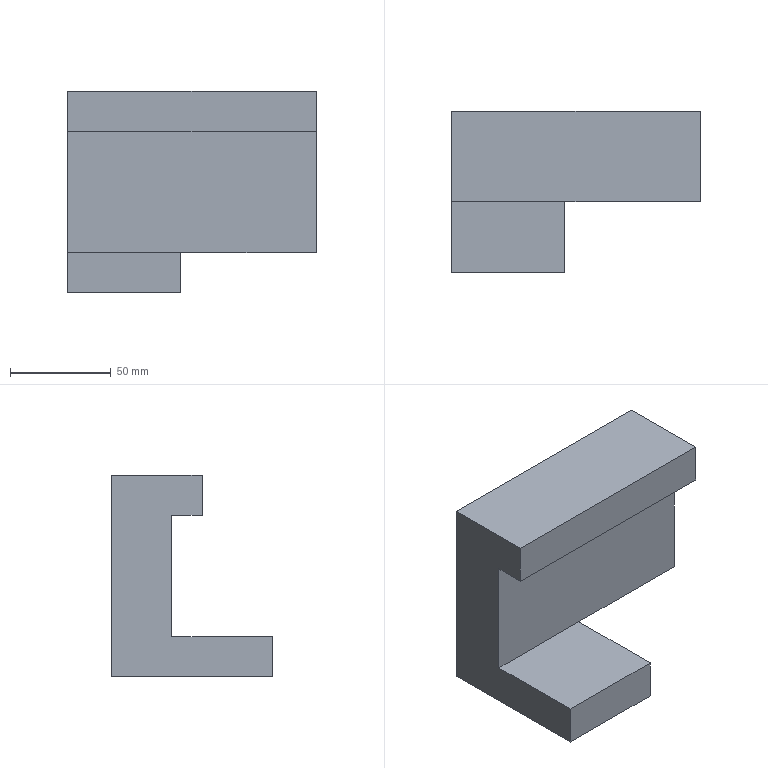Component | SolidWorks | ParallelGripperFingerA-1 | 1 solid | 12 faces | box 123 x 80 x 100 mm | volume 421700 mm3 | plane 12 | material Aviation Aluminum-7075
build123d program:
from build123d import *

# Parameters (mm, degrees)
SKETCH1_W           = 80
SKETCH1_H           = 56
BOSS_EXTRUDE1_DEPTH = 20
SKETCH2_W           = 30
SKETCH2_H           = 56
BOSS_EXTRUDE2_DEPTH = 80
SKETCH3_W           = 30
SKETCH3_H           = 80
BOSS_EXTRUDE3_DEPTH = 67
SKETCH4_W           = 20
SKETCH4_H           = 123
BOSS_EXTRUDE4_DEPTH = 15


with BuildPart() as part:
    # Sketch1 → Boss-Extrude1 (new body)
    with BuildSketch(Plane.XY):
        Rectangle(SKETCH1_W, SKETCH1_H)
    extrude(amount=BOSS_EXTRUDE1_DEPTH)

    # Sketch2 → Boss-Extrude2 (add)
    with BuildSketch(Plane.XY.offset(20)):
        with Locations((25, 0)):
            Rectangle(SKETCH2_W, SKETCH2_H)
    extrude(amount=BOSS_EXTRUDE2_DEPTH)

    # Sketch3 → Boss-Extrude3 (add)
    with BuildSketch(Plane(origin=(0, -28, 0), x_dir=(1, 0, 0), z_dir=(0, 1, 0))):
        with Locations((25, -60)):
            Rectangle(SKETCH3_W, SKETCH3_H)
    extrude(amount=-BOSS_EXTRUDE3_DEPTH)

    # Sketch4 → Boss-Extrude4 (add)
    with BuildSketch(Plane.ZY.offset(-10)):
        with Locations((90, -33.5)):
            Rectangle(SKETCH4_W, SKETCH4_H)
    extrude(amount=BOSS_EXTRUDE4_DEPTH)


solid = part.part

# Placed as in the assembly
solid = solid.moved(Location((-80.87, -240.626, 497.215), (0, 0, 90)))
STEP:
#1=CARTESIAN_POINT('',(-4.286,-9.08,22.725));
#2=VERTEX_POINT('',#1);
#3=CARTESIAN_POINT('',(0.5563,-9.08,22.725));
#4=VERTEX_POINT('',#3);
#5=CARTESIAN_POINT('',(0.5563,-9.08,22.725));
#6=DIRECTION('',(1.,0.,0.));
#7=VECTOR('',#6,39.37);
#8=LINE('',#5,#7);
#9=EDGE_CURVE('',#2,#4,#8,.T.);
#10=ORIENTED_EDGE('',*,*,#9,.F.);
#11=CARTESIAN_POINT('',(-4.286,-9.08,20.363));
#12=VERTEX_POINT('',#11);
#13=CARTESIAN_POINT('',(-4.286,-9.08,23.512));
#14=DIRECTION('',(0.,0.,-1.));
#15=VECTOR('',#14,39.37);
#16=LINE('',#13,#15);
#17=EDGE_CURVE('',#2,#12,#16,.T.);
#18=ORIENTED_EDGE('',*,*,#17,.T.);
#19=CARTESIAN_POINT('',(-2.081,-9.08,20.363));
#20=VERTEX_POINT('',#19);
#21=CARTESIAN_POINT('',(-4.286,-9.08,20.363));
#22=DIRECTION('',(1.,0.,0.));
#23=VECTOR('',#22,39.37);
#24=LINE('',#21,#23);
#25=EDGE_CURVE('',#12,#20,#24,.T.);
#26=ORIENTED_EDGE('',*,*,#25,.T.);
#27=CARTESIAN_POINT('',(0.5563,-9.08,20.363));
#28=VERTEX_POINT('',#27);
#29=CARTESIAN_POINT('',(0.5563,-9.08,20.363));
#30=DIRECTION('',(-1.,-0.,0.));
#31=VECTOR('',#30,39.37);
#32=LINE('',#29,#31);
#33=EDGE_CURVE('',#28,#20,#32,.T.);
#34=ORIENTED_EDGE('',*,*,#33,.F.);
#35=CARTESIAN_POINT('',(0.5563,-9.08,20.363));
#36=DIRECTION('',(0.,0.,1.));
#37=VECTOR('',#36,39.37);
#38=LINE('',#35,#37);
#39=EDGE_CURVE('',#28,#4,#38,.T.);
#40=ORIENTED_EDGE('',*,*,#39,.T.);
#41=EDGE_LOOP('',(#10,#18,#26,#34,#40));
#42=FACE_OUTER_BOUND('',#41,.T.);
#43=CARTESIAN_POINT('',(-4.286,-9.08,23.512));
#44=DIRECTION('',(-0.,1.,0.));
#45=DIRECTION('',(-1.,-0.,0.));
#46=AXIS2_PLACEMENT_3D('',#43,#44,#45);
#47=PLANE('',#46);
#48=ADVANCED_FACE('',(#42),#47,.F.);
#49=CARTESIAN_POINT('',(-4.286,-11.048,19.575));
#50=VERTEX_POINT('',#49);
#51=CARTESIAN_POINT('',(-2.081,-11.048,19.575));
#52=VERTEX_POINT('',#51);
#53=CARTESIAN_POINT('',(-2.081,-11.048,19.575));
#54=DIRECTION('',(1.,-0.,0.));
#55=VECTOR('',#54,39.37);
#56=LINE('',#53,#55);
#57=EDGE_CURVE('',#50,#52,#56,.T.);
#58=ORIENTED_EDGE('',*,*,#57,.T.);
#59=CARTESIAN_POINT('',(-2.081,-11.048,20.363));
#60=VERTEX_POINT('',#59);
#61=CARTESIAN_POINT('',(-2.081,-11.048,20.363));
#62=DIRECTION('',(0.,0.,-1.));
#63=VECTOR('',#62,39.37);
#64=LINE('',#61,#63);
#65=EDGE_CURVE('',#60,#52,#64,.T.);
#66=ORIENTED_EDGE('',*,*,#65,.F.);
#67=CARTESIAN_POINT('',(-4.286,-11.048,20.363));
#68=VERTEX_POINT('',#67);
#69=CARTESIAN_POINT('',(-2.081,-11.048,20.363));
#70=DIRECTION('',(1.,-0.,0.));
#71=VECTOR('',#70,39.37);
#72=LINE('',#69,#71);
#73=EDGE_CURVE('',#68,#60,#72,.T.);
#74=ORIENTED_EDGE('',*,*,#73,.F.);
#75=CARTESIAN_POINT('',(-4.286,-11.048,20.363));
#76=DIRECTION('',(0.,0.,-1.));
#77=VECTOR('',#76,39.37);
#78=LINE('',#75,#77);
#79=EDGE_CURVE('',#68,#50,#78,.T.);
#80=ORIENTED_EDGE('',*,*,#79,.T.);
#81=EDGE_LOOP('',(#58,#66,#74,#80));
#82=FACE_OUTER_BOUND('',#81,.T.);
#83=CARTESIAN_POINT('',(-2.081,-11.048,20.363));
#84=DIRECTION('',(0.,1.,0.));
#85=DIRECTION('',(0.,0.,-1.));
#86=AXIS2_PLACEMENT_3D('',#83,#84,#85);
#87=PLANE('',#86);
#88=ADVANCED_FACE('',(#82),#87,.F.);
#89=CARTESIAN_POINT('',(-2.081,-7.899,20.363));
#90=VERTEX_POINT('',#89);
#91=CARTESIAN_POINT('',(-2.081,-7.899,19.575));
#92=VERTEX_POINT('',#91);
#93=CARTESIAN_POINT('',(-2.081,-7.899,20.363));
#94=DIRECTION('',(0.,0.,-1.));
#95=VECTOR('',#94,39.37);
#96=LINE('',#93,#95);
#97=EDGE_CURVE('',#90,#92,#96,.T.);
#98=ORIENTED_EDGE('',*,*,#97,.F.);
#99=CARTESIAN_POINT('',(-2.081,-9.08,20.363));
#100=DIRECTION('',(0.,-1.,0.));
#101=VECTOR('',#100,39.37);
#102=LINE('',#99,#101);
#103=EDGE_CURVE('',#90,#20,#102,.T.);
#104=ORIENTED_EDGE('',*,*,#103,.T.);
#105=CARTESIAN_POINT('',(-2.081,-7.899,20.363));
#106=DIRECTION('',(-0.,1.,0.));
#107=VECTOR('',#106,39.37);
#108=LINE('',#105,#107);
#109=EDGE_CURVE('',#60,#20,#108,.T.);
#110=ORIENTED_EDGE('',*,*,#109,.F.);
#111=ORIENTED_EDGE('',*,*,#65,.T.);
#112=CARTESIAN_POINT('',(-2.081,-7.899,19.575));
#113=DIRECTION('',(-0.,1.,0.));
#114=VECTOR('',#113,39.37);
#115=LINE('',#112,#114);
#116=EDGE_CURVE('',#52,#92,#115,.T.);
#117=ORIENTED_EDGE('',*,*,#116,.T.);
#118=EDGE_LOOP('',(#98,#104,#110,#111,#117));
#119=FACE_OUTER_BOUND('',#118,.T.);
#120=CARTESIAN_POINT('',(-2.081,-7.899,20.363));
#121=DIRECTION('',(-1.,-0.,0.));
#122=DIRECTION('',(0.,-1.,0.));
#123=AXIS2_PLACEMENT_3D('',#120,#121,#122);
#124=PLANE('',#123);
#125=ADVANCED_FACE('',(#119),#124,.F.);
#126=CARTESIAN_POINT('',(-4.286,-7.899,19.575));
#127=VERTEX_POINT('',#126);
#128=CARTESIAN_POINT('',(-2.081,-7.899,19.575));
#129=DIRECTION('',(-1.,0.,0.));
#130=VECTOR('',#129,39.37);
#131=LINE('',#128,#130);
#132=EDGE_CURVE('',#92,#127,#131,.T.);
#133=ORIENTED_EDGE('',*,*,#132,.T.);
#134=CARTESIAN_POINT('',(-4.286,-7.899,23.512));
#135=VERTEX_POINT('',#134);
#136=CARTESIAN_POINT('',(-4.286,-7.899,20.363));
#137=DIRECTION('',(0.,0.,-1.));
#138=VECTOR('',#137,39.37);
#139=LINE('',#136,#138);
#140=EDGE_CURVE('',#135,#127,#139,.T.);
#141=ORIENTED_EDGE('',*,*,#140,.F.);
#142=CARTESIAN_POINT('',(0.5563,-7.899,23.512));
#143=VERTEX_POINT('',#142);
#144=CARTESIAN_POINT('',(-4.286,-7.899,23.512));
#145=DIRECTION('',(-1.,0.,0.));
#146=VECTOR('',#145,39.37);
#147=LINE('',#144,#146);
#148=EDGE_CURVE('',#143,#135,#147,.T.);
#149=ORIENTED_EDGE('',*,*,#148,.F.);
#150=CARTESIAN_POINT('',(0.5563,-7.899,20.363));
#151=VERTEX_POINT('',#150);
#152=CARTESIAN_POINT('',(0.5563,-7.899,20.363));
#153=DIRECTION('',(0.,0.,-1.));
#154=VECTOR('',#153,39.37);
#155=LINE('',#152,#154);
#156=EDGE_CURVE('',#143,#151,#155,.T.);
#157=ORIENTED_EDGE('',*,*,#156,.T.);
#158=CARTESIAN_POINT('',(0.5563,-7.899,20.363));
#159=DIRECTION('',(-1.,-0.,0.));
#160=VECTOR('',#159,39.37);
#161=LINE('',#158,#160);
#162=EDGE_CURVE('',#151,#90,#161,.T.);
#163=ORIENTED_EDGE('',*,*,#162,.T.);
#164=ORIENTED_EDGE('',*,*,#97,.T.);
#165=EDGE_LOOP('',(#133,#141,#149,#157,#163,#164));
#166=FACE_OUTER_BOUND('',#165,.T.);
#167=CARTESIAN_POINT('',(-2.081,-7.899,20.363));
#168=DIRECTION('',(-0.,-1.,0.));
#169=DIRECTION('',(0.,0.,1.));
#170=AXIS2_PLACEMENT_3D('',#167,#168,#169);
#171=PLANE('',#170);
#172=ADVANCED_FACE('',(#166),#171,.F.);
#173=CARTESIAN_POINT('',(-4.286,-7.899,19.575));
#174=DIRECTION('',(0.,-1.,0.));
#175=VECTOR('',#174,39.37);
#176=LINE('',#173,#175);
#177=EDGE_CURVE('',#127,#50,#176,.T.);
#178=ORIENTED_EDGE('',*,*,#177,.T.);
#179=ORIENTED_EDGE('',*,*,#79,.F.);
#180=CARTESIAN_POINT('',(-4.286,-7.899,20.363));
#181=DIRECTION('',(0.,-1.,0.));
#182=VECTOR('',#181,39.37);
#183=LINE('',#180,#182);
#184=EDGE_CURVE('',#12,#68,#183,.T.);
#185=ORIENTED_EDGE('',*,*,#184,.F.);
#186=ORIENTED_EDGE('',*,*,#17,.F.);
#187=CARTESIAN_POINT('',(-4.286,-9.67,22.725));
#188=VERTEX_POINT('',#187);
#189=CARTESIAN_POINT('',(-4.286,-9.67,22.725));
#190=DIRECTION('',(-0.,1.,0.));
#191=VECTOR('',#190,39.37);
#192=LINE('',#189,#191);
#193=EDGE_CURVE('',#188,#2,#192,.T.);
#194=ORIENTED_EDGE('',*,*,#193,.F.);
#195=CARTESIAN_POINT('',(-4.286,-9.67,23.512));
#196=VERTEX_POINT('',#195);
#197=CARTESIAN_POINT('',(-4.286,-9.67,23.512));
#198=DIRECTION('',(0.,0.,-1.));
#199=VECTOR('',#198,39.37);
#200=LINE('',#197,#199);
#201=EDGE_CURVE('',#196,#188,#200,.T.);
#202=ORIENTED_EDGE('',*,*,#201,.F.);
#203=CARTESIAN_POINT('',(-4.286,-7.899,23.512));
#204=DIRECTION('',(0.,-1.,0.));
#205=VECTOR('',#204,39.37);
#206=LINE('',#203,#205);
#207=EDGE_CURVE('',#135,#196,#206,.T.);
#208=ORIENTED_EDGE('',*,*,#207,.F.);
#209=ORIENTED_EDGE('',*,*,#140,.T.);
#210=EDGE_LOOP('',(#178,#179,#185,#186,#194,#202,#208,#209));
#211=FACE_OUTER_BOUND('',#210,.T.);
#212=CARTESIAN_POINT('',(-4.286,-7.899,20.363));
#213=DIRECTION('',(1.,0.,0.));
#214=DIRECTION('',(-0.,1.,0.));
#215=AXIS2_PLACEMENT_3D('',#212,#213,#214);
#216=PLANE('',#215);
#217=ADVANCED_FACE('',(#211),#216,.F.);
#218=ORIENTED_EDGE('',*,*,#25,.F.);
#219=ORIENTED_EDGE('',*,*,#184,.T.);
#220=ORIENTED_EDGE('',*,*,#73,.T.);
#221=ORIENTED_EDGE('',*,*,#109,.T.);
#222=EDGE_LOOP('',(#218,#219,#220,#221));
#223=FACE_OUTER_BOUND('',#222,.T.);
#224=CARTESIAN_POINT('',(-3.184,-9.473,20.363));
#225=DIRECTION('',(0.,0.,1.));
#226=DIRECTION('',(0.,1.,0.));
#227=AXIS2_PLACEMENT_3D('',#224,#225,#226);
#228=PLANE('',#227);
#229=ADVANCED_FACE('',(#223),#228,.T.);
#230=ORIENTED_EDGE('',*,*,#57,.F.);
#231=ORIENTED_EDGE('',*,*,#177,.F.);
#232=ORIENTED_EDGE('',*,*,#132,.F.);
#233=ORIENTED_EDGE('',*,*,#116,.F.);
#234=EDGE_LOOP('',(#230,#231,#232,#233));
#235=FACE_OUTER_BOUND('',#234,.T.);
#236=CARTESIAN_POINT('',(-3.184,-9.473,19.575));
#237=DIRECTION('',(0.,0.,1.));
#238=DIRECTION('',(0.,1.,0.));
#239=AXIS2_PLACEMENT_3D('',#236,#237,#238);
#240=PLANE('',#239);
#241=ADVANCED_FACE('',(#235),#240,.F.);
#242=ORIENTED_EDGE('',*,*,#148,.T.);
#243=ORIENTED_EDGE('',*,*,#207,.T.);
#244=CARTESIAN_POINT('',(0.5563,-9.67,23.512));
#245=VERTEX_POINT('',#244);
#246=CARTESIAN_POINT('',(0.5563,-9.67,23.512));
#247=DIRECTION('',(-1.,-0.,0.));
#248=VECTOR('',#247,39.37);
#249=LINE('',#246,#248);
#250=EDGE_CURVE('',#245,#196,#249,.T.);
#251=ORIENTED_EDGE('',*,*,#250,.F.);
#252=CARTESIAN_POINT('',(0.5563,-9.08,23.512));
#253=DIRECTION('',(-0.,1.,0.));
#254=VECTOR('',#253,39.37);
#255=LINE('',#252,#254);
#256=EDGE_CURVE('',#245,#143,#255,.T.);
#257=ORIENTED_EDGE('',*,*,#256,.T.);
#258=EDGE_LOOP('',(#242,#243,#251,#257));
#259=FACE_OUTER_BOUND('',#258,.T.);
#260=CARTESIAN_POINT('',(-3.184,-9.473,23.512));
#261=DIRECTION('',(0.,0.,-1.));
#262=DIRECTION('',(-0.,-1.,0.));
#263=AXIS2_PLACEMENT_3D('',#260,#261,#262);
#264=PLANE('',#263);
#265=ADVANCED_FACE('',(#259),#264,.F.);
#266=ORIENTED_EDGE('',*,*,#103,.F.);
#267=ORIENTED_EDGE('',*,*,#162,.F.);
#268=CARTESIAN_POINT('',(0.5563,-9.08,20.363));
#269=DIRECTION('',(0.,-1.,0.));
#270=VECTOR('',#269,39.37);
#271=LINE('',#268,#270);
#272=EDGE_CURVE('',#151,#28,#271,.T.);
#273=ORIENTED_EDGE('',*,*,#272,.T.);
#274=ORIENTED_EDGE('',*,*,#33,.T.);
#275=EDGE_LOOP('',(#266,#267,#273,#274));
#276=FACE_OUTER_BOUND('',#275,.T.);
#277=CARTESIAN_POINT('',(0.5563,-9.08,20.363));
#278=DIRECTION('',(0.,0.,-1.));
#279=DIRECTION('',(-0.,-1.,0.));
#280=AXIS2_PLACEMENT_3D('',#277,#278,#279);
#281=PLANE('',#280);
#282=ADVANCED_FACE('',(#276),#281,.T.);
#283=ORIENTED_EDGE('',*,*,#39,.F.);
#284=ORIENTED_EDGE('',*,*,#272,.F.);
#285=ORIENTED_EDGE('',*,*,#156,.F.);
#286=ORIENTED_EDGE('',*,*,#256,.F.);
#287=CARTESIAN_POINT('',(0.5563,-9.67,22.725));
#288=VERTEX_POINT('',#287);
#289=CARTESIAN_POINT('',(0.5563,-9.67,23.512));
#290=DIRECTION('',(0.,0.,1.));
#291=VECTOR('',#290,39.37);
#292=LINE('',#289,#291);
#293=EDGE_CURVE('',#288,#245,#292,.T.);
#294=ORIENTED_EDGE('',*,*,#293,.F.);
#295=CARTESIAN_POINT('',(0.5563,-9.67,22.725));
#296=DIRECTION('',(-0.,1.,0.));
#297=VECTOR('',#296,39.37);
#298=LINE('',#295,#297);
#299=EDGE_CURVE('',#288,#4,#298,.T.);
#300=ORIENTED_EDGE('',*,*,#299,.T.);
#301=EDGE_LOOP('',(#283,#284,#285,#286,#294,#300));
#302=FACE_OUTER_BOUND('',#301,.T.);
#303=CARTESIAN_POINT('',(0.5563,-9.473,19.575));
#304=DIRECTION('',(-1.,-0.,0.));
#305=DIRECTION('',(0.,-1.,0.));
#306=AXIS2_PLACEMENT_3D('',#303,#304,#305);
#307=PLANE('',#306);
#308=ADVANCED_FACE('',(#302),#307,.F.);
#309=ORIENTED_EDGE('',*,*,#9,.T.);
#310=ORIENTED_EDGE('',*,*,#299,.F.);
#311=CARTESIAN_POINT('',(0.5563,-9.67,22.725));
#312=DIRECTION('',(1.,0.,0.));
#313=VECTOR('',#312,39.37);
#314=LINE('',#311,#313);
#315=EDGE_CURVE('',#188,#288,#314,.T.);
#316=ORIENTED_EDGE('',*,*,#315,.F.);
#317=ORIENTED_EDGE('',*,*,#193,.T.);
#318=EDGE_LOOP('',(#309,#310,#316,#317));
#319=FACE_OUTER_BOUND('',#318,.T.);
#320=CARTESIAN_POINT('',(0.5563,-9.67,22.725));
#321=DIRECTION('',(0.,0.,1.));
#322=DIRECTION('',(0.,1.,0.));
#323=AXIS2_PLACEMENT_3D('',#320,#321,#322);
#324=PLANE('',#323);
#325=ADVANCED_FACE('',(#319),#324,.F.);
#326=ORIENTED_EDGE('',*,*,#250,.T.);
#327=ORIENTED_EDGE('',*,*,#201,.T.);
#328=ORIENTED_EDGE('',*,*,#315,.T.);
#329=ORIENTED_EDGE('',*,*,#293,.T.);
#330=EDGE_LOOP('',(#326,#327,#328,#329));
#331=FACE_OUTER_BOUND('',#330,.T.);
#332=CARTESIAN_POINT('',(-3.184,-9.67,19.575));
#333=DIRECTION('',(0.,-1.,0.));
#334=DIRECTION('',(1.,0.,0.));
#335=AXIS2_PLACEMENT_3D('',#332,#333,#334);
#336=PLANE('',#335);
#337=ADVANCED_FACE('',(#331),#336,.T.);
#338=CLOSED_SHELL('',(#48,#88,#125,#172,#217,#229,#241,#265,#282,#308,#325,#337));
#339=MANIFOLD_SOLID_BREP('',#338);
#340=CARTESIAN_POINT('',(0.,0.,0.));
#341=DIRECTION('',(0.,0.,1.));
#342=DIRECTION('',(1.,0.,0.));
#343=AXIS2_PLACEMENT_3D('',#340,#341,#342);
#344=(LENGTH_UNIT()NAMED_UNIT(*)SI_UNIT($,.METRE.));
#345=LENGTH_MEASURE_WITH_UNIT(LENGTH_MEASURE(0.0254),#344);
#346=DIMENSIONAL_EXPONENTS(1.,0.,0.,0.,0.,0.,0.);
#347=(CONVERSION_BASED_UNIT('',#345)LENGTH_UNIT()NAMED_UNIT(#346));
#348=UNCERTAINTY_MEASURE_WITH_UNIT(LENGTH_MEASURE(0.00001),#347,'','');
#349=(NAMED_UNIT(*)PLANE_ANGLE_UNIT()SI_UNIT($,.RADIAN.));
#350=(NAMED_UNIT(*)SI_UNIT($,.STERADIAN.)SOLID_ANGLE_UNIT());
#351=(GEOMETRIC_REPRESENTATION_CONTEXT(3)GLOBAL_UNCERTAINTY_ASSIGNED_CONTEXT((#348))GLOBAL_UNIT_ASSIGNED_CONTEXT((#347,#349,#350))REPRESENTATION_CONTEXT('',''));
#352=ADVANCED_BREP_SHAPE_REPRESENTATION('',(#339,#343),#351);
#353=COLOUR_RGB('',0.7922,0.8196,0.9333);
#354=FILL_AREA_STYLE_COLOUR('',#353);
#355=FILL_AREA_STYLE('',(#354));
#356=SURFACE_STYLE_FILL_AREA(#355);
#357=SURFACE_SIDE_STYLE('',(#356));
#358=SURFACE_STYLE_USAGE(.BOTH.,#357);
#359=PRESENTATION_STYLE_ASSIGNMENT((#358));
#360=STYLED_ITEM('',(#359),#339);
#361=PRESENTATION_LAYER_ASSIGNMENT('','',(#360));
#362=(LENGTH_UNIT()NAMED_UNIT(*)SI_UNIT($,.METRE.));
#363=LENGTH_MEASURE_WITH_UNIT(LENGTH_MEASURE(0.0254),#362);
#364=DIMENSIONAL_EXPONENTS(1.,0.,0.,0.,0.,0.,0.);
#365=(CONVERSION_BASED_UNIT('',#363)LENGTH_UNIT()NAMED_UNIT(#364));
#366=UNCERTAINTY_MEASURE_WITH_UNIT(LENGTH_MEASURE(0.00001),#365,'','');
#367=(NAMED_UNIT(*)PLANE_ANGLE_UNIT()SI_UNIT($,.RADIAN.));
#368=(NAMED_UNIT(*)SI_UNIT($,.STERADIAN.)SOLID_ANGLE_UNIT());
#369=(GEOMETRIC_REPRESENTATION_CONTEXT(3)GLOBAL_UNCERTAINTY_ASSIGNED_CONTEXT((#366))GLOBAL_UNIT_ASSIGNED_CONTEXT((#365,#367,#368))REPRESENTATION_CONTEXT('',''));
#370=MECHANICAL_DESIGN_GEOMETRIC_PRESENTATION_REPRESENTATION('',(#360),#369);